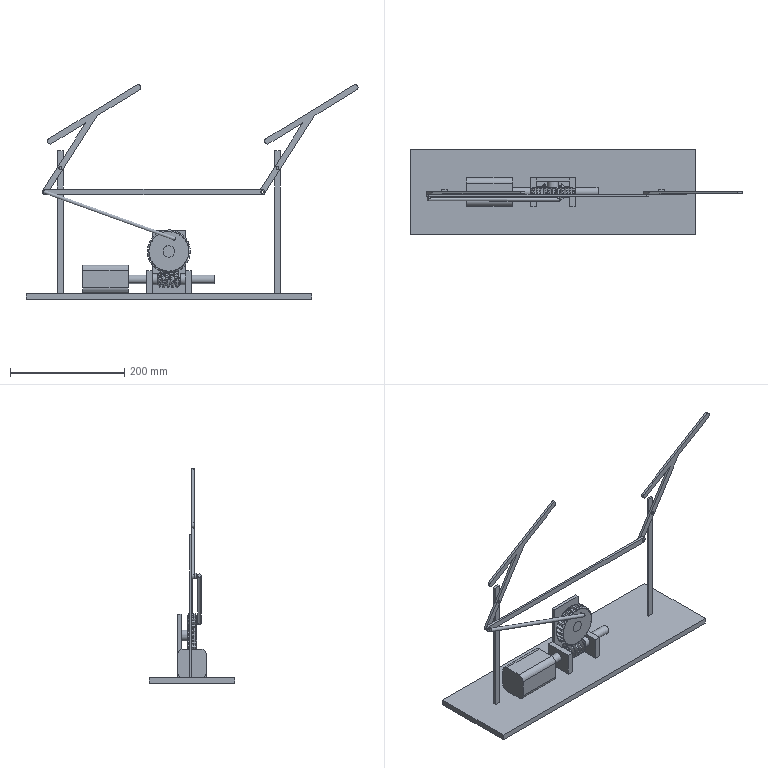Assembly | NX | mm | 8 component files | 8 solids | 275 faces | box 580.94 x 150 x 375.77 mm | volume 1193602 mm3 | spline 87 | plane 67 | cylinder 62 | cone 59 | commonest cylinder face diameters 75 x28 5 x11 10 x8 20 x6 15 x5 19 x2 6 x1 30 x1
Bill of materials:
unnamed part 1 | 1 |  | Long, slender flat bar with rounded (semicircular) ends and one small through hole near each end.
unnamed part 2 | 1 |  | Cylindrical shaft with a larger-diameter helical threaded section in the middle, short collars on each side of it, and plain cylindrical ends.
unnamed part 3 | 1 |  | Toothed disc (gear-like wheel) with about 26 teeth, a central round bore, and one small hole offset from the center.
unnamed part 4 | 1 |  | Rectangular block with rounded long edges (rounded-square cross-section) and a round hole on one end face.
unnamed part 5 | 1 |  | Round rod bent into a shallow U (staple shape): a long straight section with a short perpendicular leg at each end, both pointing the same way.
unnamed part 6 | 1 |  | Flat rectangular base plate holding two tall thin vertical posts near its ends and a cluster of blocks in the middle: an upright plate with a projecting cylindrical boss, and small blocks with holes.
unnamed part 7 | 2 |  | Flat bar shaped like a Y (or tilted T): a long straight bar with rounded ends, joined by a second straight arm at an acute angle. The arm has a hole at its free end and another partway along.
Mates:
1. fix | base_plate 1 component
2. touch align | motor 1 face | base_plate 1 face
3. center | motor 1 face | motor 1 face | base_plate 1 face | base_plate 1 face
4. center | worm 1 face | worm 1 face | base_plate 1
5. touch align | worm 1 face | motor 1 face
6. touch align | worm 1 face | motor 1 face
7. concentric | link_2 1 edge | worm_wheel 1 edge
8. touch align | link_2 1 face | link 1 face
9. touch align | wiper 2 face | link 1 face
10. touch align | wiper 2 face | link_2 1 face
11. touch align | base_plate 1 face | wiper 2 face
12. concentric | base_plate 1 edge | worm_wheel 1 edge
13. parallel | link 1 face | base_plate 1 face
14. touch align | wiper 1 face | base_plate 1 face
15. touch align | link_2 1 face | wiper 2 face
16. parallel | wiper 1 face | wiper 2 face